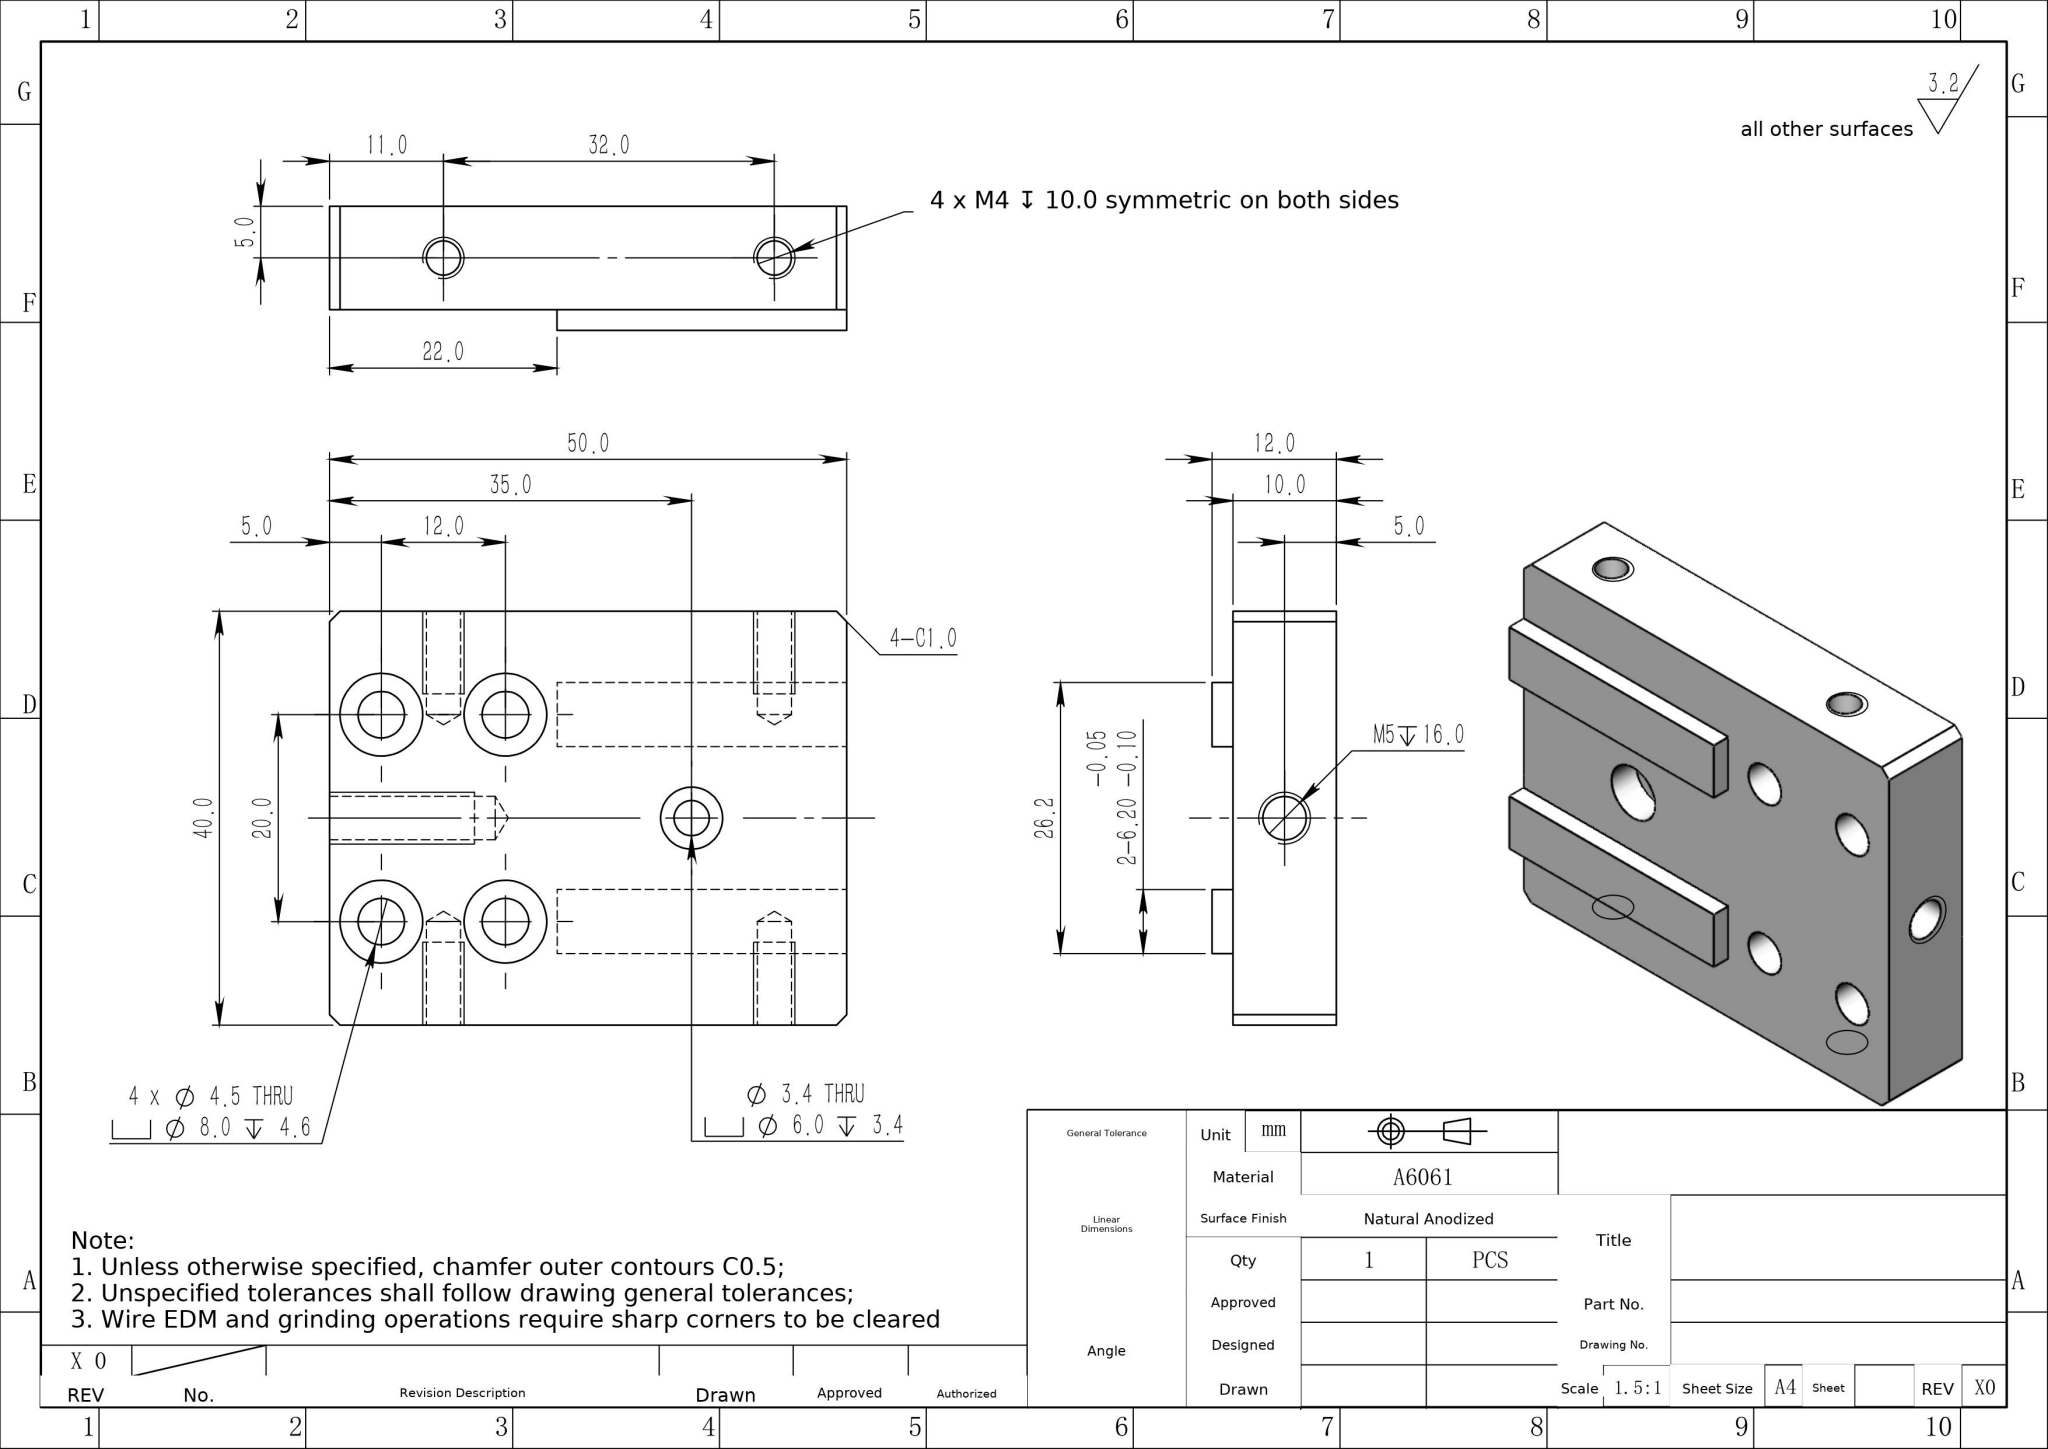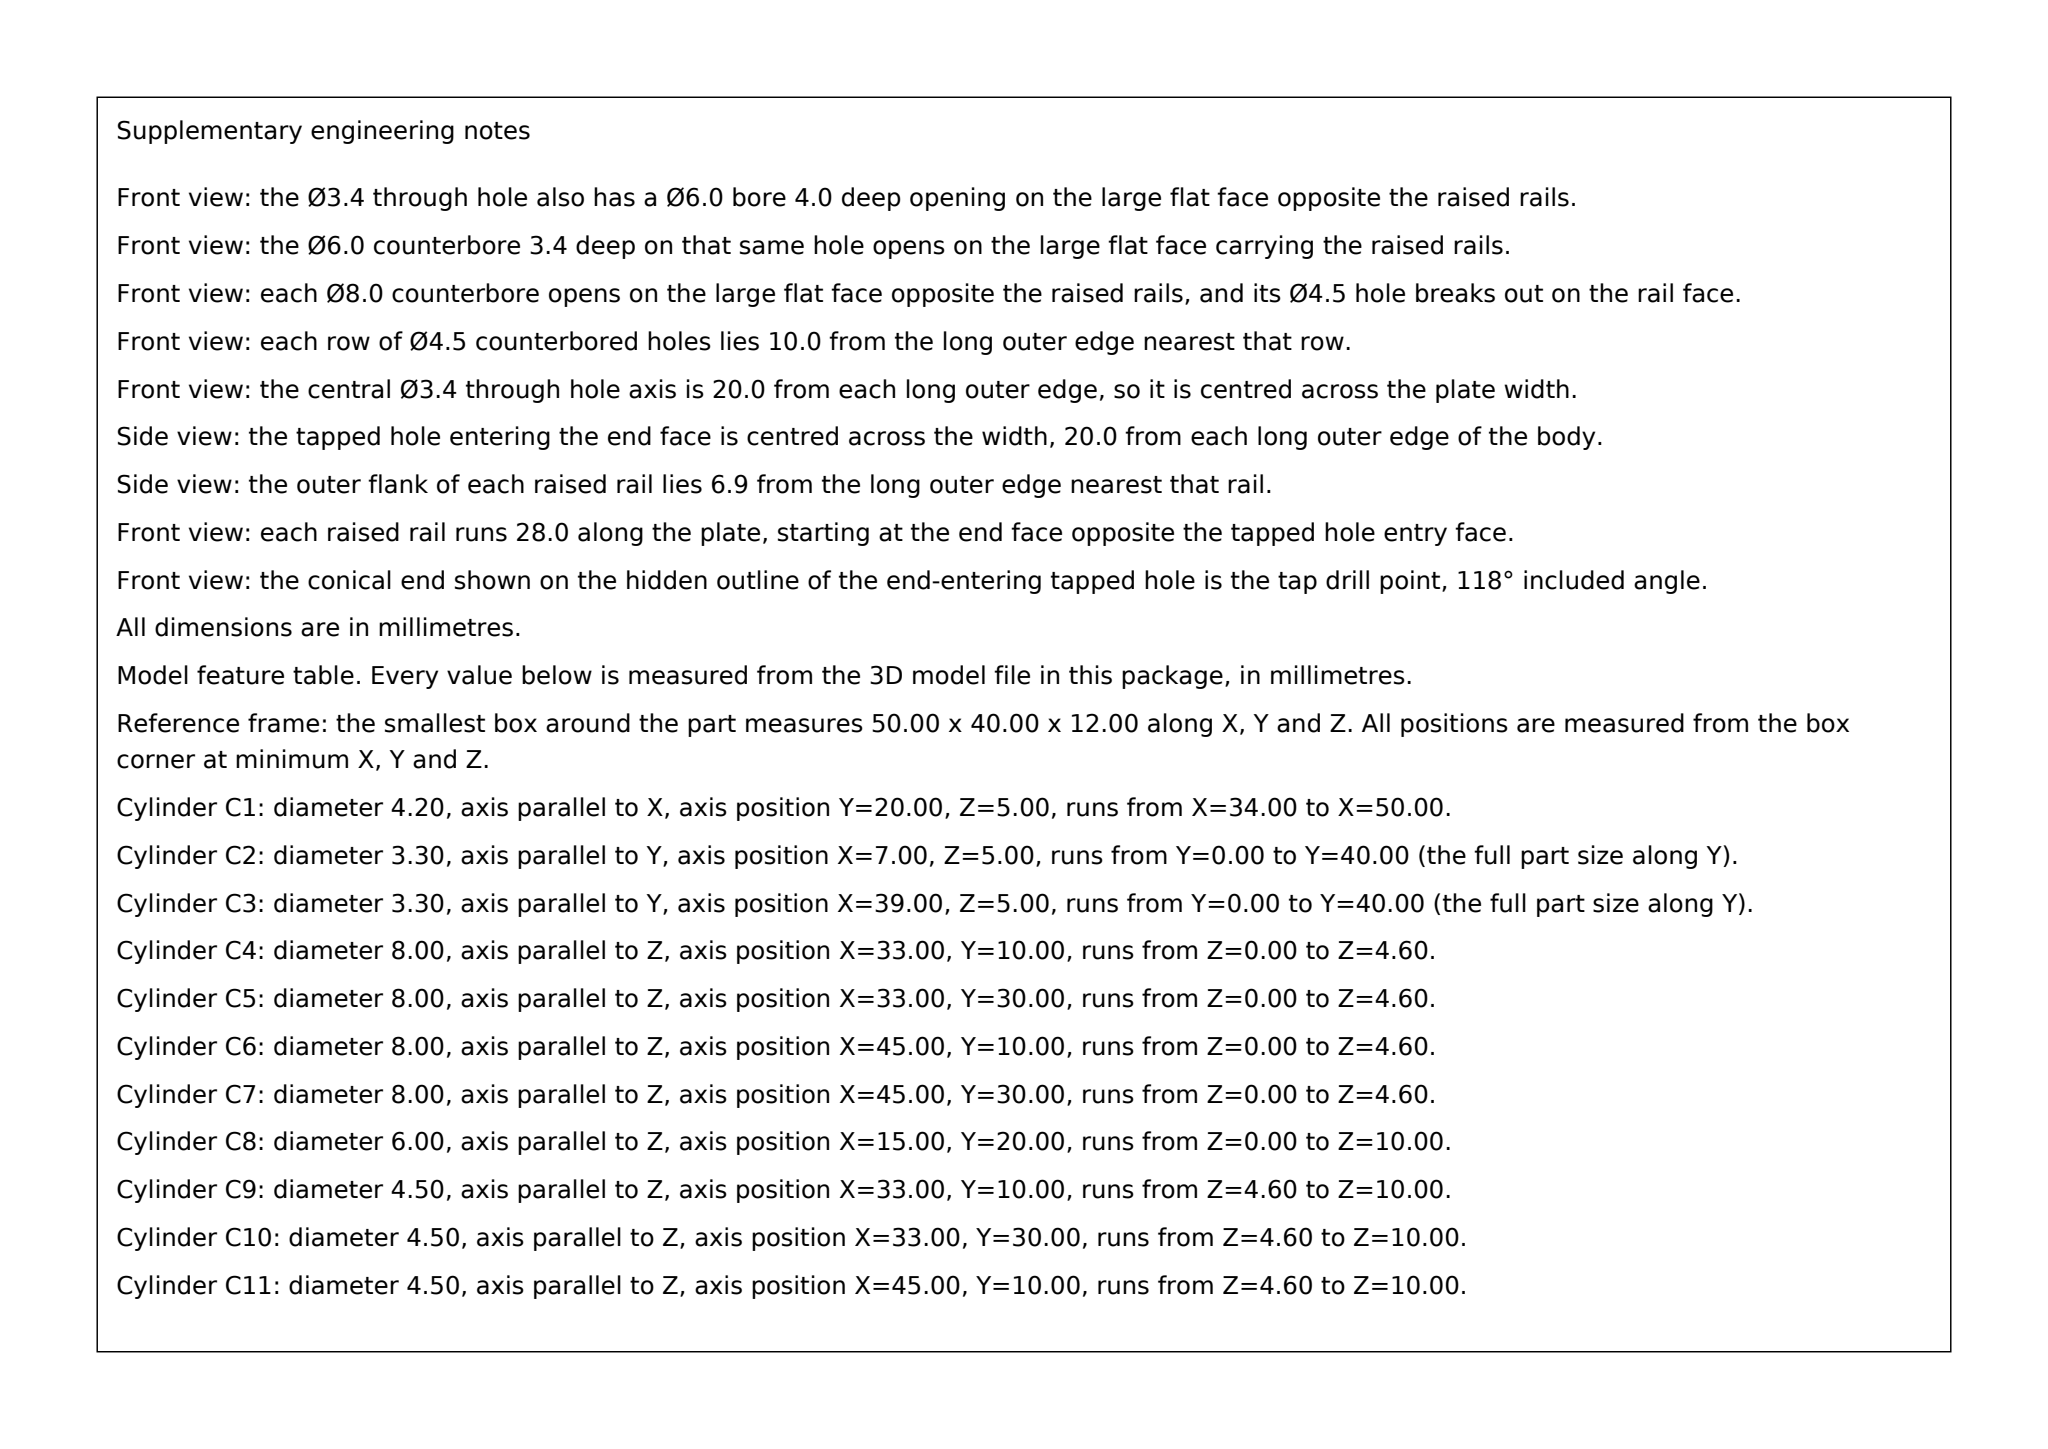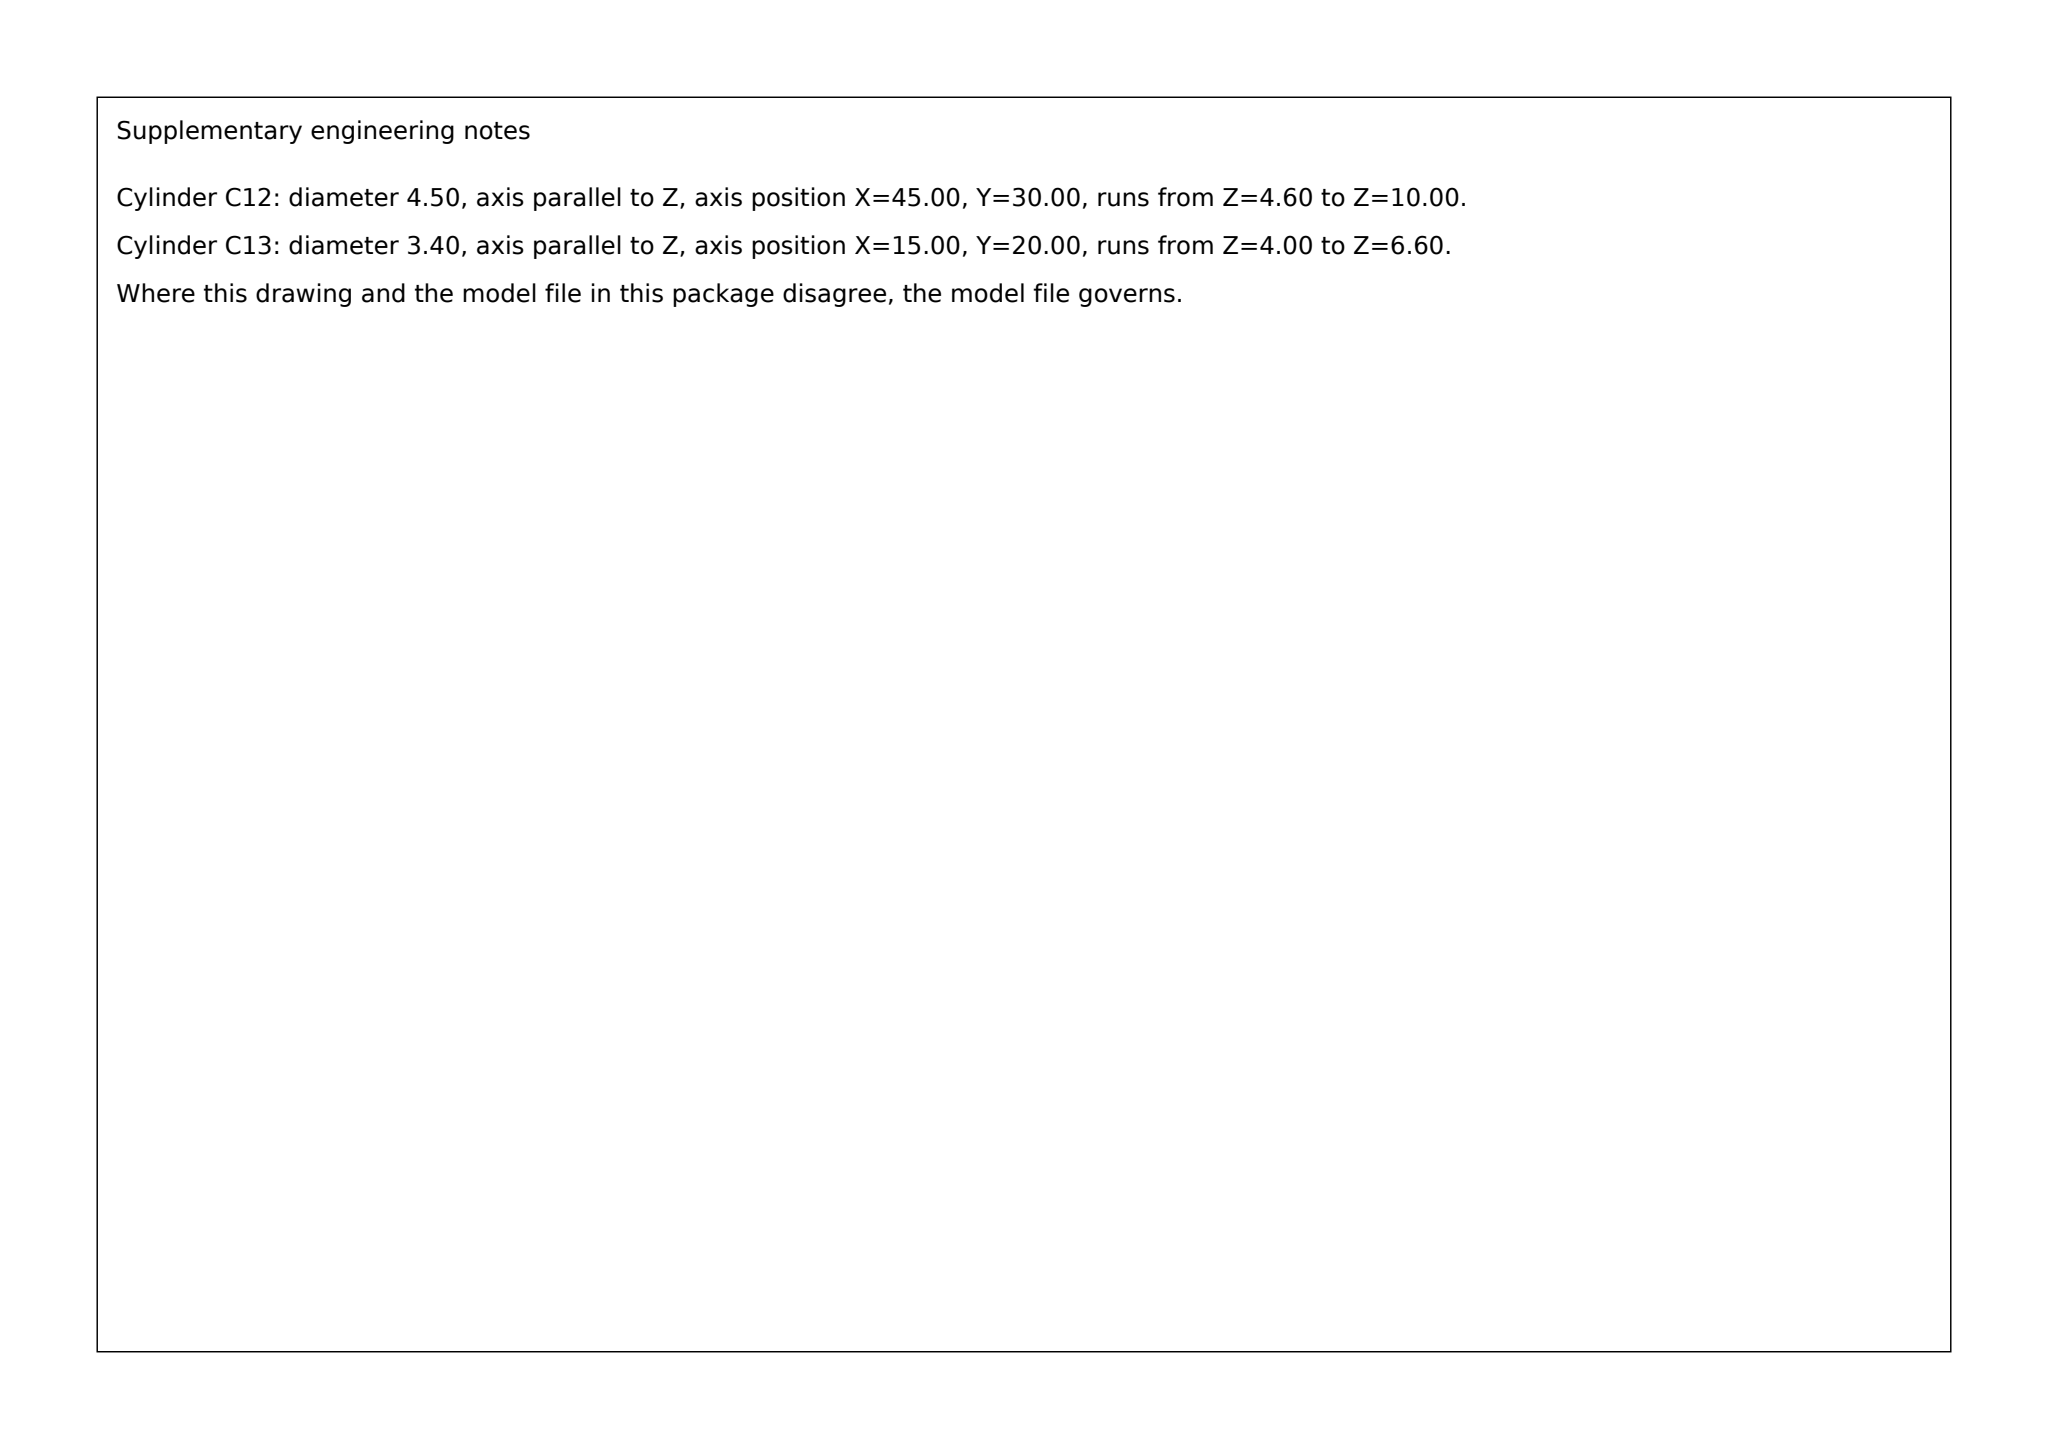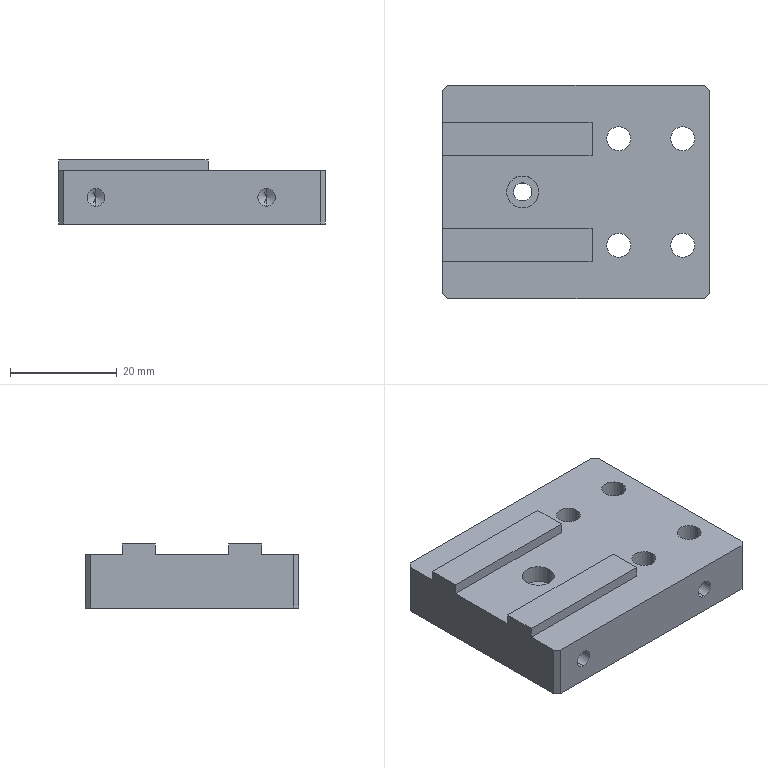Part | SolidWorks | mm | material A6061 | 1 solid | 66 faces | box 50 x 40 x 12 mm | volume 18592 mm3 | cylinder 32 | plane 24 | cone 10 | commonest cylinder face diameters 3.3 x8 8 x8 4.5 x8 6 x4 4.2 x2 3.4 x2
Drawing notes:
Ø3.4 THRU: CBORE Ø6.0 DP 3.4 THIS FACE, CBORE Ø6.0 DP 4.0 OPPOSITE FACE | from the solid: Ø3.4 bore z=4.0-6.6 at (x15,y20); Ø6.0 bore z=6.6-10.0 (3.4 deep from z=10 face) and Ø6.0 bore z=0-4.0 (4.0 deep from z=0 face), flat faces at z=4.0 and z=6.6
build123d program:
from build123d import *

# Parameters (mm, degrees)
SKETCH1_W                                            = 50
SKETCH1_H                                            = 40
BOSS_EXTRUDE1_DEPTH                                  = 6
HOLE_SIZE_ACCORDING_TO_TYPE_3_OF_HEXAGON_D           = 4.5
HOLE_SIZE_ACCORDING_TO_TYPE_3_OF_HEXAGON_CBORE_D     = 8
HOLE_SIZE_ACCORDING_TO_TYPE_3_OF_HEXAGON_CBORE_DEPTH = 4.6
SKETCH10_W                                           = 50
SKETCH10_H                                           = 6.9
SKETCH10_H_2                                         = 13.8
CUT_EXTRUDE3_DEPTH                                   = 2
SKETCH13_R                                           = 3
CUT_EXTRUDE4_DEPTH                                   = 4
HOLE_SIZE_ACCORDING_TO_TYPE_3_OF_HEX_2_D             = 3.4
HOLE_SIZE_ACCORDING_TO_TYPE_3_OF_HEX_2_CBORE_D       = 6
HOLE_SIZE_ACCORDING_TO_TYPE_3_OF_HEX_2_CBORE_DEPTH   = 3.4
M5_TAPPED_HOLE1_D                                    = 4.2
M5_TAPPED_HOLE1_DEPTH                                = 16
M5_TAPPED_HOLE1_TIP                                  = 1.262
SKETCH20_W                                           = 22
SKETCH20_H                                           = 40
CUT_EXTRUDE5_DEPTH                                   = 2
M4_TAPPED_HOLE1_AT_2_COUNT                           = 2
M4_TAPPED_HOLE1_AT_2_PITCH                           = 32
CHAMFER1_SIZE                                        = 1


with BuildPart() as part:
    # Sketch1 → Boss-Extrude1 (new, symmetric)
    with BuildSketch(Plane.XY):
        Rectangle(SKETCH1_W, SKETCH1_H)
    extrude(amount=BOSS_EXTRUDE1_DEPTH, both=True)

    # Hole Size_According to_Type 3 of Hexagon (through all)
    with Locations(Plane(origin=(0, 0, -6), x_dir=(-1, 0, 0), z_dir=(0, 0, -1))):
        with Locations((-20, 10), (-20, -10), (-8, 10), (-8, -10)):
            CounterBoreHole(HOLE_SIZE_ACCORDING_TO_TYPE_3_OF_HEXAGON_D / 2, HOLE_SIZE_ACCORDING_TO_TYPE_3_OF_HEXAGON_CBORE_D / 2, HOLE_SIZE_ACCORDING_TO_TYPE_3_OF_HEXAGON_CBORE_DEPTH)

    # Sketch10 → Cut-Extrude3 (cut)
    with BuildSketch(Plane.XY.offset(6)):
        with Locations((0, 16.55)):
            Rectangle(SKETCH10_W, SKETCH10_H)
        Rectangle(SKETCH10_W, SKETCH10_H_2)
        with Locations((0, -16.55)):
            Rectangle(SKETCH10_W, SKETCH10_H)
    extrude(amount=-CUT_EXTRUDE3_DEPTH, mode=Mode.SUBTRACT)

    # Sketch13 → Cut-Extrude4 (cut)
    with BuildSketch(Plane(origin=(0, 0, -6), x_dir=(-1, 0, 0), z_dir=(0, 0, -1))):
        with Locations((10, 0)):
            Circle(SKETCH13_R)
    extrude(amount=-CUT_EXTRUDE4_DEPTH, mode=Mode.SUBTRACT)

    # Hole Size_According to_Type 3 of Hex 2 (through all)
    with Locations(Plane.XY.offset(4)):
        with Locations((-10, 0)):
            CounterBoreHole(HOLE_SIZE_ACCORDING_TO_TYPE_3_OF_HEX_2_D / 2, HOLE_SIZE_ACCORDING_TO_TYPE_3_OF_HEX_2_CBORE_D / 2, HOLE_SIZE_ACCORDING_TO_TYPE_3_OF_HEX_2_CBORE_DEPTH)

    # M5 Tapped Hole1
    with Locations(Plane(origin=(25, 0, 0), x_dir=(0, 0, -1), z_dir=(1, 0, 0))):
        with Locations((1, 0)):
            Hole(M5_TAPPED_HOLE1_D / 2, depth=M5_TAPPED_HOLE1_DEPTH)
            with Locations((0, 0, -(M5_TAPPED_HOLE1_DEPTH + M5_TAPPED_HOLE1_TIP / 2))):  # 118° drill point
                Cone(0, M5_TAPPED_HOLE1_D / 2, M5_TAPPED_HOLE1_TIP, mode=Mode.SUBTRACT)

    # Sketch20 → Cut-Extrude5 (cut)
    with BuildSketch(Plane.XY.offset(6)):
        with Locations((14, 0)):
            Rectangle(SKETCH20_W, SKETCH20_H)
    extrude(amount=-CUT_EXTRUDE5_DEPTH, mode=Mode.SUBTRACT)

    # Sketch22 → M4 Tapped Hole1 (revolve, cut)
    with BuildSketch(Plane(origin=(14, -20, -1), x_dir=(0, 0, -1), z_dir=(1, 0, 0))):
        Polygon((0, 0), (0, 10.991), (1.65, 10), (1.65, 0), align=None)
    m4_tapped_hole1 = revolve(axis=Axis((14, -26.35, -1), (0, 1, 0)), mode=Mode.SUBTRACT)

    # M4 Tapped Hole1 at 2: M4 Tapped Hole1 ×2
    with Locations(*[(-i * M4_TAPPED_HOLE1_AT_2_PITCH, 0, 0) for i in range(1, M4_TAPPED_HOLE1_AT_2_COUNT)]):
        add(m4_tapped_hole1, mode=Mode.SUBTRACT)

    # Mirror1: M4 Tapped Hole1 across plane
    add(m4_tapped_hole1.mirror(Plane.ZX), mode=Mode.SUBTRACT)

    # Mirror1 copy 1 sketch → Mirror1 copy 1 (revolve, cut)
    with BuildSketch(Plane(origin=(-18, 20, -1), x_dir=(0, 0, -1), z_dir=(1, 0, 0))):
        Polygon((0, 0), (0, -10.991), (1.65, -10), (1.65, 0), align=None)
    revolve(axis=Axis((-18, 26.35, -1), (0, 1, 0)), mode=Mode.SUBTRACT)

    # Chamfer1
    chamfer1_edges = [part.edges().sort_by_distance(p)[0] for p in [
        (-25, 20, -1),
        (25, 20, -1),
        (25, -20, -1),
        (-25, -20, -1),
    ]]
    chamfer(chamfer1_edges, length=CHAMFER1_SIZE)


solid = part.part